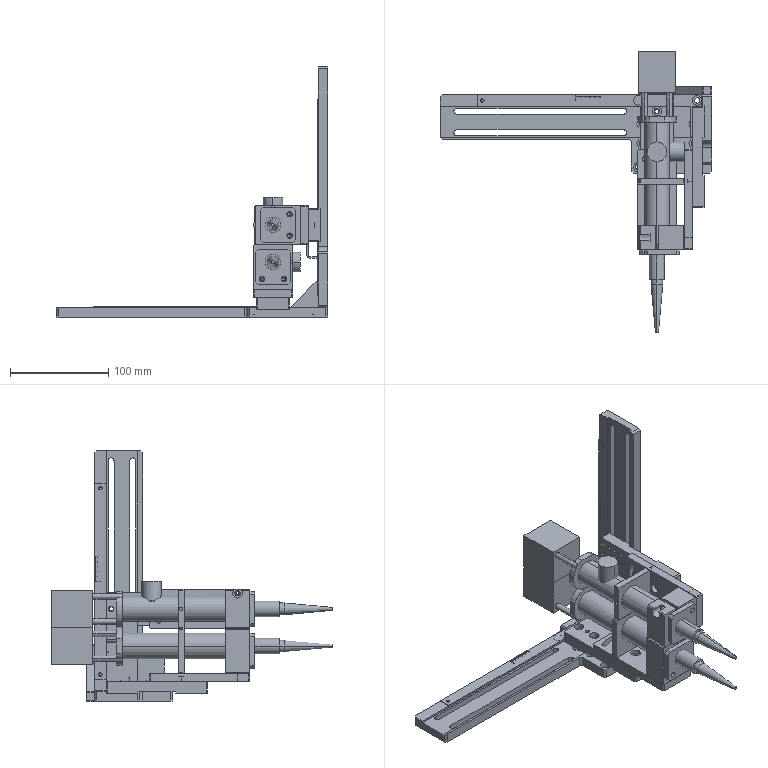Assembly | SolidWorks | mm | 18 component files | 24 solids | 820 faces | box 277 x 286 x 255 mm | volume 749260 mm3 | plane 472 | cylinder 296 | cone 52 | commonest cylinder face diameters 5.5 x62 4.2 x46 9.8 x38 6 x22 6.5 x12 5 x12 3.3 x12 7.9 x8
Bill of materials:
BLR41-L200 | 2 |  | Long, narrow, very thin flat rectangular strip with one small round through-hole near each end.
MTCTV2104DJ006-000-0038Slider | 2 |  | Elongated rectangular bar or block with a row of seven round through-holes of mixed sizes along its centerline. A shallow rectangular recess or step is cut across one face, and the outline corners are chamfered.
MTCTV2104DJ006-000-0039Trimmer | 2 |  | Rectangular flat plate with chamfered corners. It has three larger holes in a column at one end, a pair of smaller holes and a single central hole in the middle region, and a curved arc-shaped slot near the opposite end.
MTCTV2104DJ006-000-0040LimitingPart | 2 |  | Rectangular plate with chamfered corners and a large circular through-bore offset toward one side. Two small holes are drilled into one narrow edge face.
MTCTV2104DJ006-000-0041ClampBlock | 2 |  | Rectangular block with a large cylindrical through-bore and a narrow slit running from the bore to one outer face, forming a split-clamp-like geometry. A transverse hole crosses the slit, and holes are drilled into an adjacent face.
MTCTV2104DJ006-000-0042StopPart | 2 |  | Thick near-square flat plate with large corner chamfers. A large round through-hole is offset toward one side, and two smaller round through-holes sit near the opposite edge.
MTCTV2104DJ006-000-0044SlidePlate2 | 1 |  | Long, thin, L-shaped profile plate: a narrow upright section with two long parallel through-slots and a wider foot section with a small hole pattern. A stepped or recessed region runs along part of one face.
MTCTV2104DJ006-000-0045RibPlate2 | 1 |  | Flat bracket-shaped plate of uniform thickness with an angled gusset-like outline: two arms at right angles joined by a diagonal edge, each arm ending in a round through-hole.
MTCTV2104DJ006-000-0046_SheetMetalPart | 1 |  | L-shaped angle bracket made from a thin uniform-thickness sheet with a radiused bend. The tall flange has two round through-holes and chamfered top corners; the short flange is plain.
MTCTV2104DJ006-000-0043SlidePlate | 1 |  | Long flat plate with an L-shaped or offset outline: a long narrow arm with two long parallel through-slots and a thin groove line, and a wider end pad with many round holes of several sizes.
RubberHead | 2 |  | Elongated axisymmetric body: a stepped cylindrical barrel ending in a long tapered conical tip. It has a short cylindrical side boss, a flange collar at the rear, and two thin rods connecting the collar to a rectangular box-shaped block.
Mates:
1. coincident | MTCTV2104DJ006-007-0000AdjustableAssembly-1/MTCTV2104DJ006-000-0042StopPart-2 face at (3.798, -100.678, 222.447) dir (0, 1, 0) | RubberHead-2 face at (3.798, -100.678, 227.447) dir (0, -1, 0)
2. concentric | MTCTV2104DJ006-007-0000AdjustableAssembly-1/MTCTV2104DJ006-000-0041ClampBlock-2 face at (3.798, -100.678, 227.447) dir (0, 1, 0) r 13 | RubberHead-2 face at (3.798, -100.678, 227.447) dir (0, 1, 0) r 13
3. coincident | MTCTV2104DJ006-007-0000AdjustableAssembly-1/MTCTV2104DJ006-000-0043SlidePlate-1 face at (-78.702, 17.781, 181.447) dir (0, 0, 1) | MTCTV2104DJ006-000-0044SlidePlate2-2 face at (49.798, -13.219, 181.447) dir (0, 0, -1)
4. concentric | MTCTV2104DJ006-007-0000AdjustableAssembly-1/MTCTV2104DJ006-000-0043SlidePlate-1 face at (54.798, 52.281, 171.447) dir (0, 0, -1) r 4.9 | MTCTV2104DJ006-000-0044SlidePlate2-2 face at (54.798, 52.281, 181.447) dir (0, 0, -1) r 2.1
5. concentric | MTCTV2104DJ006-007-0000AdjustableAssembly-1/MTCTV2104DJ006-000-0043SlidePlate-1 face at (54.798, -7.719, 171.447) dir (0, 0, -1) r 2.75 | MTCTV2104DJ006-000-0044SlidePlate2-2 face at (54.798, -7.719, 181.447) dir (0, 0, -1) r 2.1
6. coincident | MTCTV2104DJ006-000-0044SlidePlate2-2 face at (49.798, 22.281, 307.447) dir (-1, 0, 0) | BLR41-L200-1 face at (49.798, 57.781, 193.447) dir (1, 0, 0)
7. concentric | MTCTV2104DJ006-000-0044SlidePlate2-2 face at (49.798, 51.781, 198.447) dir (-1, 0, 0) r 1.25 | BLR41-L200-1 edge at (49.298, 51.781, 198.447) dir (1, 0, 0) r 1.75
8. coincident | MTCTV2104DJ006-000-0044SlidePlate2-2 face at (51.798, 22.281, 307.447) dir (-1, 0, 0) | MTCTV2104DJ006-000-0038Slider-1 face at (51.798, -5.719, 265.447) dir (1, 0, 0)
9. coincident | MTCTV2104DJ006-000-0044SlidePlate2-2 face at (51.798, 45.781, 181.447) dir (0, -1, 0) | MTCTV2104DJ006-000-0038Slider-1 face at (39.798, 45.781, 248.447) dir (0, 1, 0)
10. coincident | MTCTV2104DJ006-000-0038Slider-1 face at (39.798, -5.719, 265.447) dir (-1, 0, 0) | MTCTV2104DJ006-000-0039Trimmer-1 face at (39.798, -29.678, 265.447) dir (1, 0, 0)
11. parallel | MTCTV2104DJ006-000-0038Slider-1 face at (39.798, 45.781, 248.447) dir (0, 1, 0) | MTCTV2104DJ006-000-0039Trimmer-1 face at (39.798, 1.322, 265.447) dir (0, 1, 0)
12. coincident | MTCTV2104DJ006-000-0039Trimmer-1 face at (31.798, -29.678, 265.447) dir (-1, 0, 0) | MTCTV2104DJ006-000-0041ClampBlock-1 face at (31.798, -88.178, 265.447) dir (1, 0, 0)
13. concentric | MTCTV2104DJ006-000-0039Trimmer-1 face at (31.798, -88.178, 281.447) dir (-1, 0, 0) r 3.25 | MTCTV2104DJ006-000-0041ClampBlock-1 face at (31.798, -88.178, 281.447) dir (1, 0, 0) r 2.5
14. concentric | MTCTV2104DJ006-000-0039Trimmer-1 face at (31.798, -88.178, 249.447) dir (-1, 0, 0) r 3.25 | MTCTV2104DJ006-000-0041ClampBlock-1 face at (31.798, -88.178, 249.447) dir (1, 0, 0) r 2.5
15. coincident | MTCTV2104DJ006-000-0039Trimmer-1 face at (31.798, -29.678, 265.447) dir (-1, 0, 0) | MTCTV2104DJ006-000-0040LimitingPart-1 face at (31.798, -27.678, 245.447) dir (1, 0, 0)
16. concentric | MTCTV2104DJ006-000-0039Trimmer-1 face at (39.798, -30.678, 249.447) dir (1, 0, 0) r 3.95 | MTCTV2104DJ006-000-0040LimitingPart-1 face at (31.798, -30.678, 249.447) dir (1, 0, 0) r 1.65
17. concentric | MTCTV2104DJ006-000-0039Trimmer-1 face at (39.798, -30.678, 281.447) dir (1, 0, 0) r 2.25 | MTCTV2104DJ006-000-0040LimitingPart-1 face at (31.798, -30.678, 281.447) dir (1, 0, 0) r 1.65
18. coincident | MTCTV2104DJ006-000-0041ClampBlock-1 face at (-14.202, -100.678, 245.447) dir (0, -1, 0) | RubberHead-3 face at (3.798, -100.678, 265.447) dir (0, -1, 0)
19. concentric | MTCTV2104DJ006-000-0041ClampBlock-1 face at (3.798, -100.678, 265.447) dir (0, 1, 0) r 13 | RubberHead-3 face at (3.798, -100.678, 265.447) dir (0, 1, 0) r 13
20. parallel | MTCTV2104DJ006-000-0044SlidePlate2-2 face at (49.798, 22.281, 307.447) dir (-1, 0, 0) | RubberHead-3 face at (22.798, 101.322, 284.447) dir (1, 0, 0)
21. coincident | MTCTV2104DJ006-000-0041ClampBlock-1 face at (-14.202, -100.678, 245.447) dir (0, -1, 0) | MTCTV2104DJ006-000-0042StopPart-1 face at (8.798, -100.678, 265.447) dir (0, 1, 0)
22. concentric | RubberHead-3 face at (3.798, -100.678, 265.447) dir (0, 1, 0) r 8 | MTCTV2104DJ006-000-0042StopPart-1 face at (3.798, -100.678, 265.447) dir (0, -1, 0) r 8
23. concentric | MTCTV2104DJ006-000-0041ClampBlock-1 face at (20.798, -100.678, 254.447) dir (0, -1, 0) r 2.1 | MTCTV2104DJ006-000-0042StopPart-1 face at (20.798, -100.678, 254.447) dir (0, -1, 0) r 2.75
24. coincident | MTCTV2104DJ006-000-0044SlidePlate2-2 face at (49.798, 57.781, 181.447) dir (0, 1, 0) | MTCTV2104DJ006-000-0045RibPlate2-1 face at (1.798, 57.781, 171.447) dir (0, -1, 0)
25. concentric | MTCTV2104DJ006-007-0000AdjustableAssembly-1/MTCTV2104DJ006-000-0043SlidePlate-1 face at (9.798, 57.781, 176.447) dir (0, 1, 0) r 2.1 | MTCTV2104DJ006-000-0045RibPlate2-1 face at (9.798, 65.781, 176.447) dir (0, 1, 0) r 2.75
26. concentric | MTCTV2104DJ006-000-0044SlidePlate2-2 face at (54.798, 57.781, 221.447) dir (0, 1, 0) r 2.1 | MTCTV2104DJ006-000-0045RibPlate2-1 face at (54.798, 65.781, 221.447) dir (0, 1, 0) r 2.75
27. coincident | MTCTV2104DJ006-007-0000AdjustableAssembly-1/MTCTV2104DJ006-000-0040LimitingPart-2 face at (-16.202, -27.678, 245.447) dir (0, 0, 1) | MTCTV2104DJ006-000-0040LimitingPart-1 face at (-14.202, -27.678, 245.447) dir (0, 0, -1)
28. coincident | MTCTV2104DJ006-000-0038Slider-1 face at (39.798, -5.719, 265.447) dir (-1, 0, 0) | MTCTV2104DJ006-000-0046_SheetMetalPart-1 face at (39.798, 29.781, 254.197) dir (1, 0, 0)
29. concentric | MTCTV2104DJ006-000-0038Slider-1 face at (39.798, 18.781, 265.447) dir (-1, 0, 0) r 2.1 | MTCTV2104DJ006-000-0046_SheetMetalPart-1 face at (38.298, 18.781, 265.447) dir (-1, 0, 0) r 2.75
30. concentric | MTCTV2104DJ006-000-0038Slider-1 face at (39.798, 40.781, 265.447) dir (-1, 0, 0) r 2.1 | MTCTV2104DJ006-000-0046_SheetMetalPart-1 face at (38.298, 40.781, 265.447) dir (-1, 0, 0) r 2.75
31. concentric | MTCTV2104DJ006-000-0044SlidePlate2-2 face at (49.798, 51.781, 388.447) dir (-1, 0, 0) r 1.25 | BLR41-L200-1 face at (49.298, 51.781, 388.447) dir (1, 0, 0) r 1.75
32. concentric | MTCTV2104DJ006-000-0038Slider-1 face at (39.798, -40.719, 265.447) dir (-1, 0, 0) r 2.1 | MTCTV2104DJ006-000-0039Trimmer-1 face at (31.798, -40.719, 265.447) dir (-1, 0, 0) r 5
33. parallel | MTCTV2104DJ006-007-0000AdjustableAssembly-1/MTCTV2104DJ006-000-0043SlidePlate-1 face at (-217.202, 57.781, 171.447) dir (0, 1, 0) | assembly plane at (0, 0, 0) dir (0, 1, 0)
34. parallel | MTCTV2104DJ006-000-0044SlidePlate2-2 face at (51.798, 22.281, 307.447) dir (-1, 0, 0) | assembly plane at (0, 0, 0) dir (1, 0, 0)
35. coincident | MTCTV2104DJ006-000-0038Slider-2 face at (9.19, -17.619, 200.197) dir (1, 0, 0) | MTCTV2104DJ006-000-0039Trimmer-2 face at (9.19, -41.578, 200.197) dir (-1, 0, 0)
36. coincident | MTCTV2104DJ006-000-0041ClampBlock-2 face at (63.19, -112.578, 220.197) dir (0, -1, 0) | MTCTV2104DJ006-000-0042StopPart-2 face at (40.19, -112.578, 200.197) dir (0, 1, 0)
37. concentric | MTCTV2104DJ006-000-0041ClampBlock-2 face at (28.19, -112.578, 189.197) dir (0, -1, 0) r 2.1 | MTCTV2104DJ006-000-0042StopPart-2 face at (28.19, -112.578, 189.197) dir (0, -1, 0) r 2.75
38. concentric | MTCTV2104DJ006-000-0041ClampBlock-2 face at (28.19, -112.578, 211.197) dir (0, -1, 0) r 2.1 | MTCTV2104DJ006-000-0042StopPart-2 face at (28.19, -112.578, 211.197) dir (0, -1, 0) r 2.75
39. coincident | MTCTV2104DJ006-000-0043SlidePlate-1 face at (-0.81, 5.881, 282.697) dir (1, 0, 0) | BLR41-L200-1 face at (-0.81, 45.881, 383.197) dir (-1, 0, 0)
40. concentric | MTCTV2104DJ006-000-0043SlidePlate-1 face at (-10.81, 39.881, 378.197) dir (-1, 0, 0) r 1.25 | BLR41-L200-1 face at (-0.31, 39.881, 378.197) dir (-1, 0, 0) r 1.75
41. concentric | MTCTV2104DJ006-000-0043SlidePlate-1 face at (-10.81, 39.881, 188.197) dir (-1, 0, 0) r 1.25 | BLR41-L200-1 face at (-0.31, 39.881, 188.197) dir (-1, 0, 0) r 1.75
42. coincident | MTCTV2104DJ006-000-0039Trimmer-2 face at (17.19, -41.578, 200.197) dir (1, 0, 0) | MTCTV2104DJ006-000-0041ClampBlock-2 face at (17.19, -100.078, 200.197) dir (-1, 0, 0)
43. concentric | MTCTV2104DJ006-000-0039Trimmer-2 face at (17.19, -100.078, 184.197) dir (1, 0, 0) r 3.25 | MTCTV2104DJ006-000-0041ClampBlock-2 face at (17.19, -100.078, 184.197) dir (-1, 0, 0) r 2.5
44. concentric | MTCTV2104DJ006-000-0039Trimmer-2 face at (17.19, -100.078, 216.197) dir (1, 0, 0) r 3.25 | MTCTV2104DJ006-000-0041ClampBlock-2 face at (17.19, -100.078, 216.197) dir (-1, 0, 0) r 2.5
45. coincident | MTCTV2104DJ006-000-0039Trimmer-2 face at (17.19, -41.578, 200.197) dir (1, 0, 0) | MTCTV2104DJ006-000-0040LimitingPart-2 face at (17.19, -39.578, 220.197) dir (-1, 0, 0)
46. concentric | MTCTV2104DJ006-000-0039Trimmer-2 face at (9.19, -42.578, 216.197) dir (-1, 0, 0) r 2.25 | MTCTV2104DJ006-000-0040LimitingPart-2 face at (17.19, -42.578, 216.197) dir (-1, 0, 0) r 1.65
47. concentric | MTCTV2104DJ006-000-0039Trimmer-2 face at (9.19, -42.578, 184.197) dir (-1, 0, 0) r 2.25 | MTCTV2104DJ006-000-0040LimitingPart-2 face at (17.19, -42.578, 184.197) dir (-1, 0, 0) r 1.65
48. coincident | MTCTV2104DJ006-000-0038Slider-2 face at (-2.81, -17.619, 200.197) dir (-1, 0, 0) | MTCTV2104DJ006-000-0043SlidePlate-1 face at (-2.81, 5.881, 282.697) dir (1, 0, 0)
49. concentric | MTCTV2104DJ006-000-0038Slider-2 face at (9.19, 28.881, 200.197) dir (1, 0, 0) r 2.75 | MTCTV2104DJ006-000-0043SlidePlate-1 face at (-2.81, 28.881, 200.197) dir (1, 0, 0) r 2.1
50. concentric | MTCTV2104DJ006-000-0038Slider-2 face at (9.19, 6.881, 200.197) dir (1, 0, 0) r 2.75 | MTCTV2104DJ006-000-0043SlidePlate-1 face at (-2.81, 6.881, 200.197) dir (1, 0, 0) r 2.1
51. concentric | MTCTV2104DJ006-000-0038Slider-2 face at (9.19, -52.619, 200.197) dir (1, 0, 0) r 2.1 | MTCTV2104DJ006-000-0039Trimmer-2 face at (17.19, -52.619, 200.197) dir (1, 0, 0) r 2.75
52. parallel | MTCTV2104DJ006-000-0043SlidePlate-1 face at (-0.81, 5.881, 282.697) dir (1, 0, 0) | MTCTV2104DJ006-007-0000AdjustableAssembly plane at (0, 0, 0) dir (1, 0, 0)
53. parallel | MTCTV2104DJ006-000-0043SlidePlate-1 face at (-10.81, 45.881, 421.197) dir (0, 1, 0) | MTCTV2104DJ006-007-0000AdjustableAssembly plane at (0, 0, 0) dir (0, 1, 0)